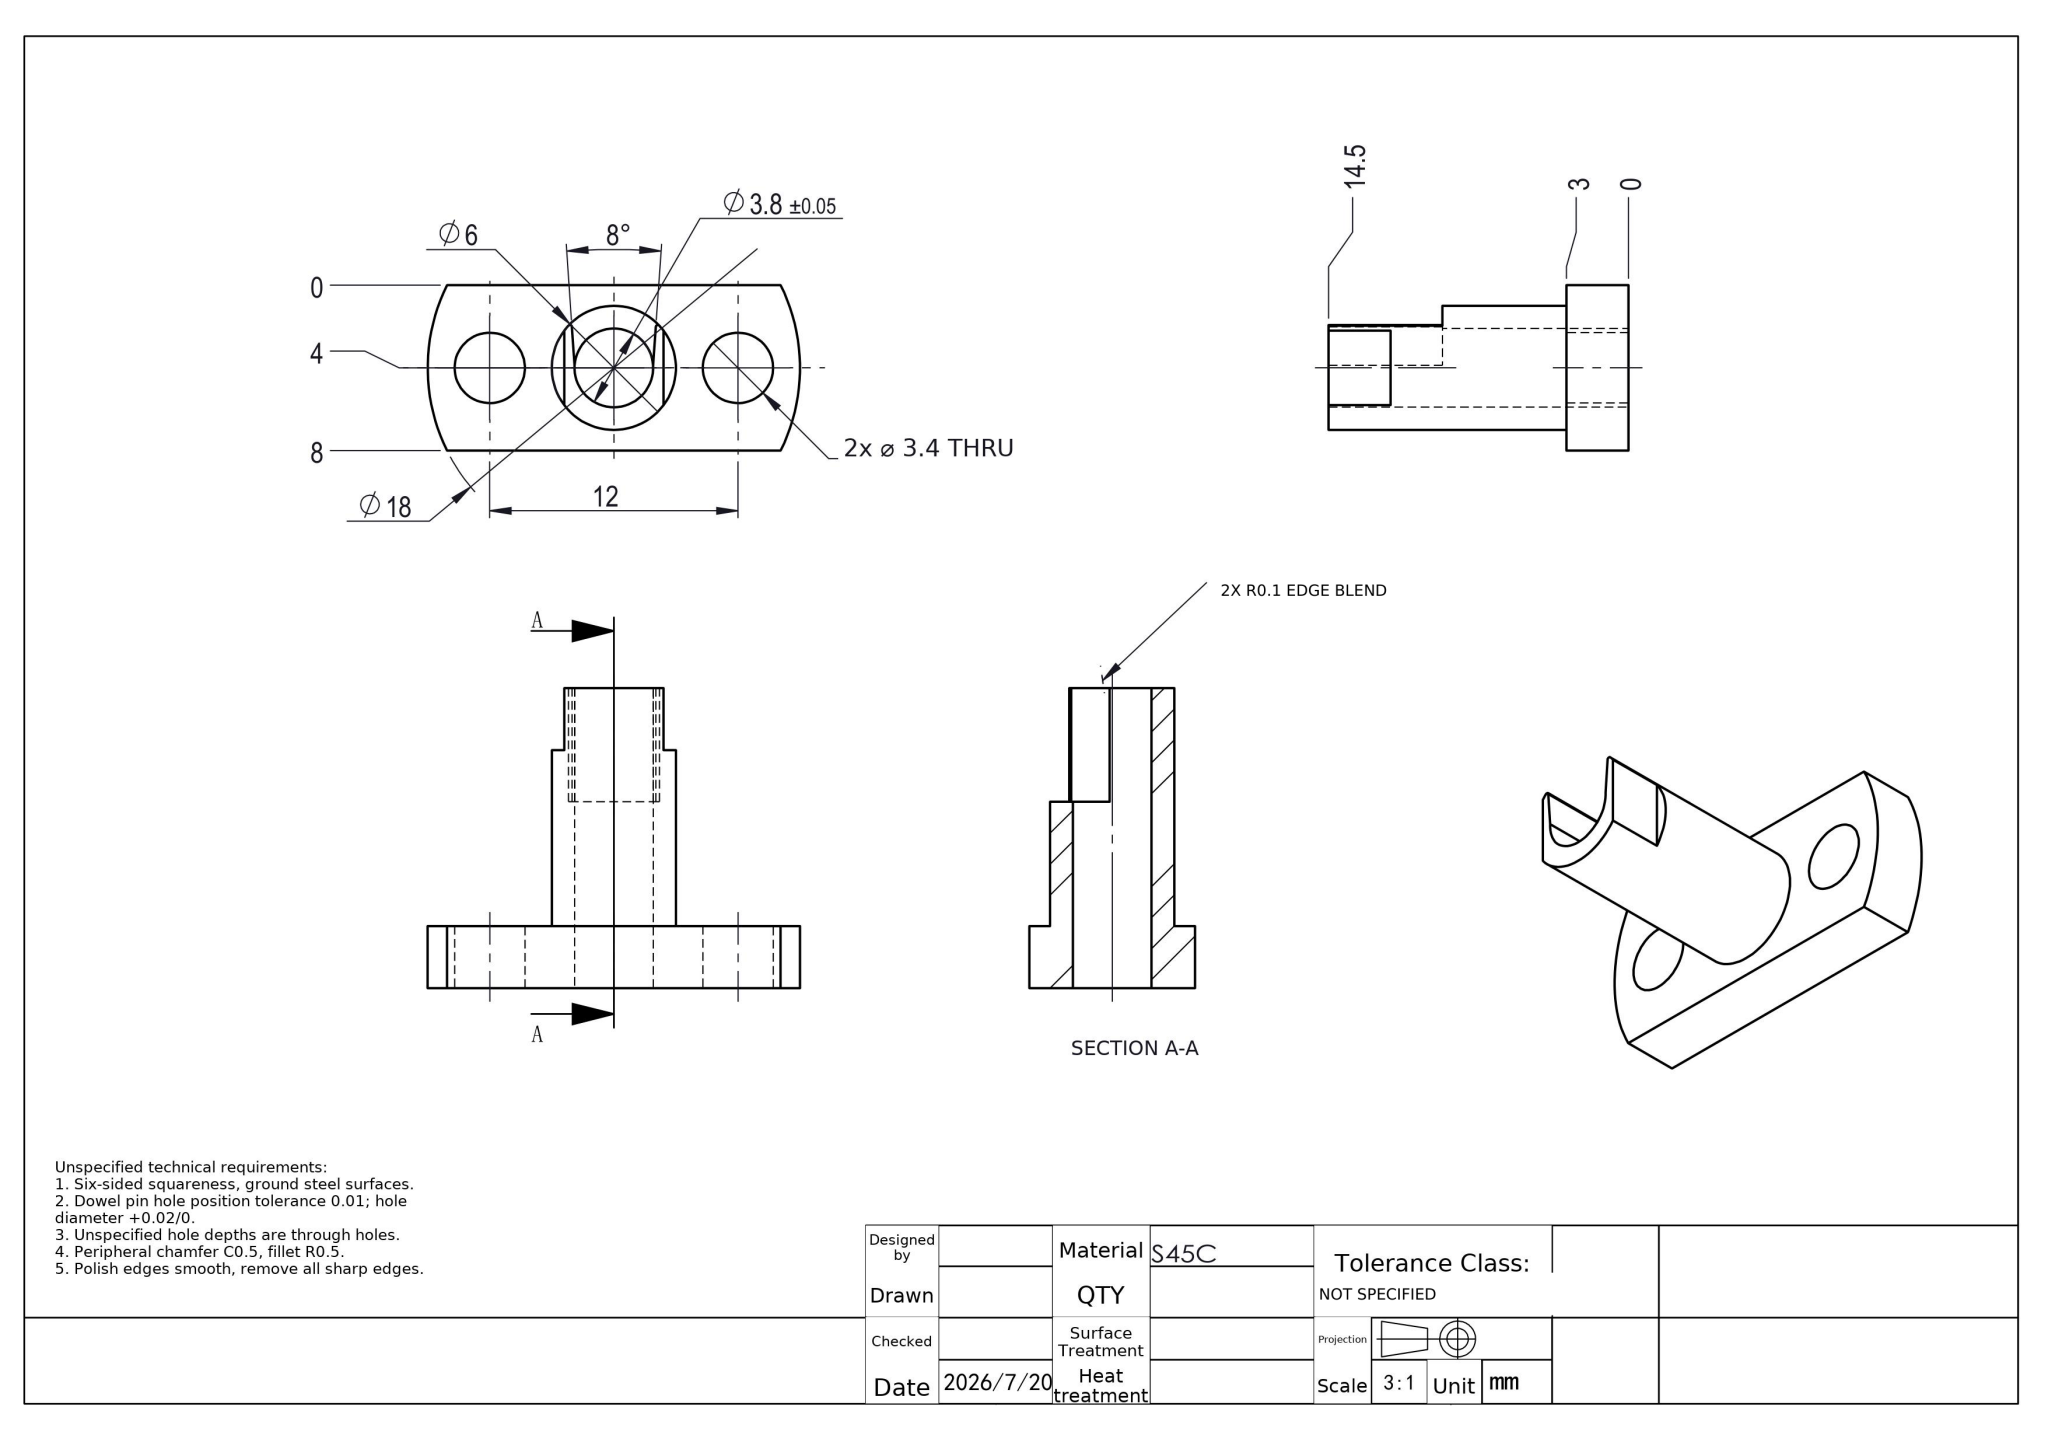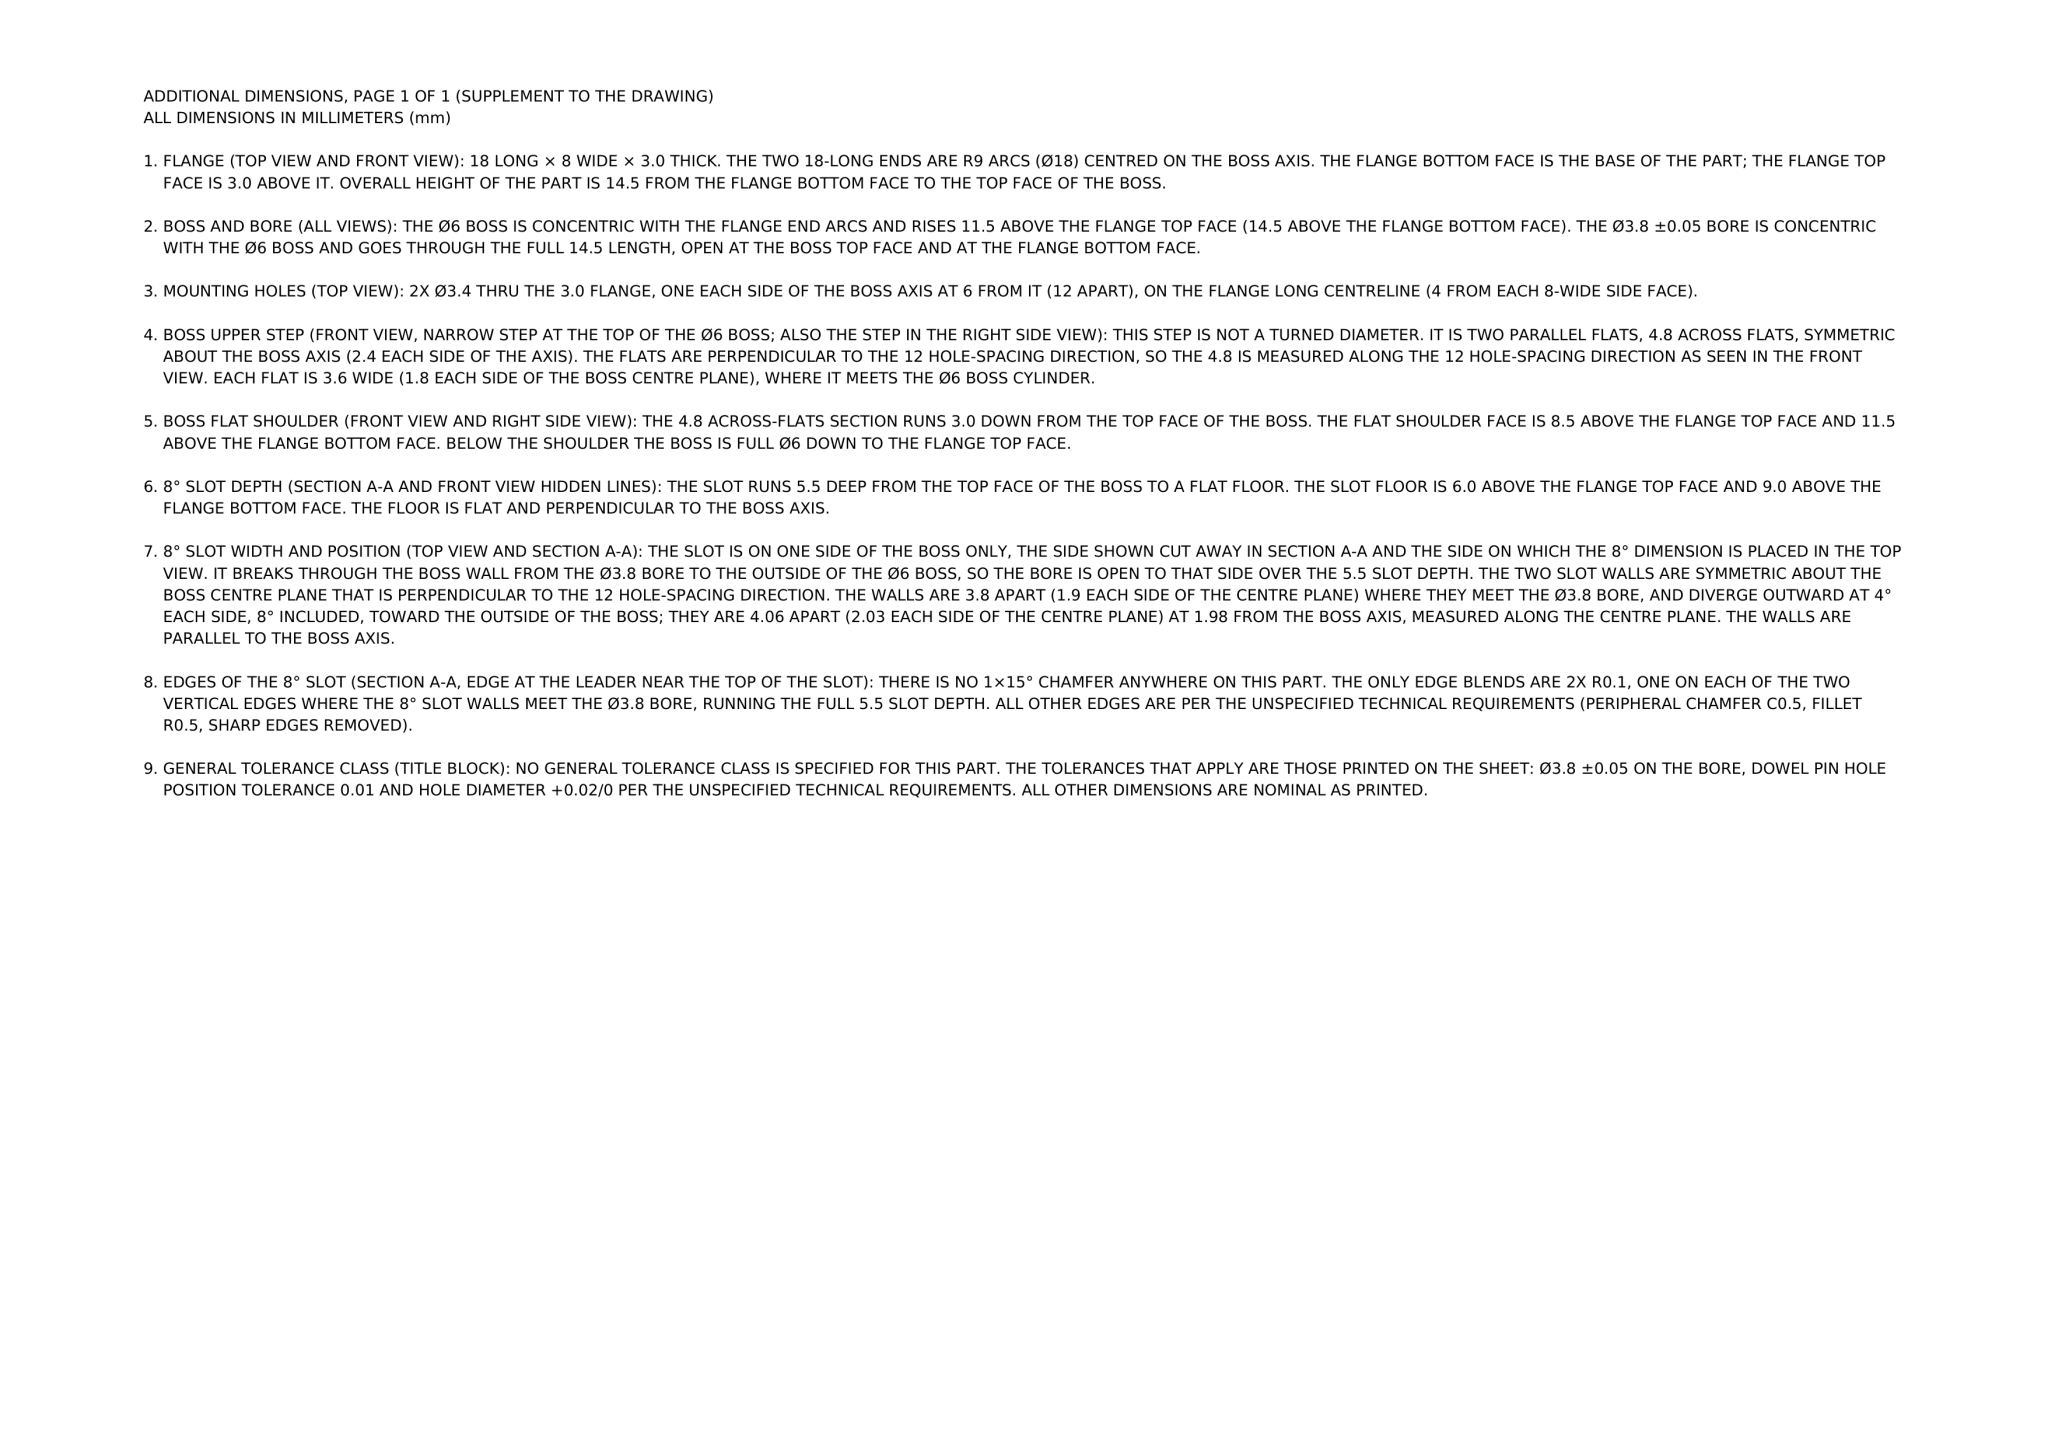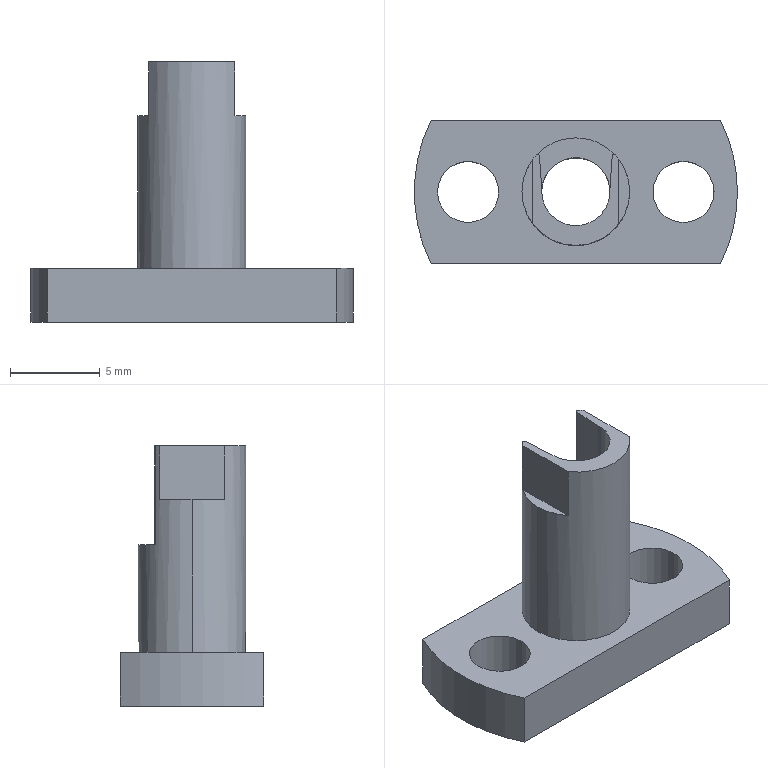Part | NX | mm | 1 solid | 25 faces | box 18 x 8 x 14.5 mm | volume 486 mm3 | cylinder 13 | plane 12 | commonest cylinder face diameters 3.4 x4 18 x3 3.8 x2 6 x2 0.2 x2
STEP:
#1=COLOUR_RGB('',0.7922,0.8196,0.9333);
#2=FILL_AREA_STYLE_COLOUR('',#1);
#3=FILL_AREA_STYLE('',(#2));
#4=SURFACE_STYLE_FILL_AREA(#3);
#5=SURFACE_SIDE_STYLE('',(#4));
#6=SURFACE_STYLE_USAGE(.BOTH.,#5);
#7=PRESENTATION_STYLE_ASSIGNMENT((#6));
#8=CARTESIAN_POINT('',(7.7,0.,0.));
#9=VERTEX_POINT('',#8);
#10=CARTESIAN_POINT('',(4.3,0.,0.));
#11=VERTEX_POINT('',#10);
#12=CARTESIAN_POINT('',(6.,0.,0.));
#13=DIRECTION('',(0.,0.,-1.));
#14=DIRECTION('',(-1.,0.,0.));
#15=AXIS2_PLACEMENT_3D('',#12,#13,#14);
#16=CIRCLE('',#15,1.7);
#17=EDGE_CURVE('',#9,#11,#16,.T.);
#18=ORIENTED_EDGE('',*,*,#17,.F.);
#19=CARTESIAN_POINT('',(7.7,0.,-3.));
#20=VERTEX_POINT('',#19);
#21=CARTESIAN_POINT('',(7.7,0.,-3.));
#22=DIRECTION('',(0.,0.,-1.));
#23=VECTOR('',#22,1000.);
#24=LINE('',#21,#23);
#25=EDGE_CURVE('',#9,#20,#24,.T.);
#26=ORIENTED_EDGE('',*,*,#25,.T.);
#27=CARTESIAN_POINT('',(4.3,0.,-3.));
#28=VERTEX_POINT('',#27);
#29=CARTESIAN_POINT('',(6.,0.,-3.));
#30=DIRECTION('',(0.,0.,-1.));
#31=DIRECTION('',(-1.,0.,0.));
#32=AXIS2_PLACEMENT_3D('',#29,#30,#31);
#33=CIRCLE('',#32,1.7);
#34=EDGE_CURVE('',#20,#28,#33,.T.);
#35=ORIENTED_EDGE('',*,*,#34,.T.);
#36=CARTESIAN_POINT('',(4.3,0.,-3.));
#37=DIRECTION('',(0.,0.,-1.));
#38=VECTOR('',#37,1000.);
#39=LINE('',#36,#38);
#40=EDGE_CURVE('',#11,#28,#39,.T.);
#41=ORIENTED_EDGE('',*,*,#40,.F.);
#42=EDGE_LOOP('',(#18,#26,#35,#41));
#43=FACE_OUTER_BOUND('',#42,.T.);
#44=CARTESIAN_POINT('',(6.,0.,-3.));
#45=DIRECTION('',(0.,0.,-1.));
#46=DIRECTION('',(-1.,0.,0.));
#47=AXIS2_PLACEMENT_3D('',#44,#45,#46);
#48=CYLINDRICAL_SURFACE('',#47,1.7);
#49=ADVANCED_FACE('',(#43),#48,.F.);
#50=CARTESIAN_POINT('',(-4.3,0.,0.));
#51=VERTEX_POINT('',#50);
#52=CARTESIAN_POINT('',(-7.7,0.,0.));
#53=VERTEX_POINT('',#52);
#54=CARTESIAN_POINT('',(-6.,0.,0.));
#55=DIRECTION('',(0.,0.,-1.));
#56=DIRECTION('',(-1.,0.,0.));
#57=AXIS2_PLACEMENT_3D('',#54,#55,#56);
#58=CIRCLE('',#57,1.7);
#59=EDGE_CURVE('',#51,#53,#58,.T.);
#60=ORIENTED_EDGE('',*,*,#59,.F.);
#61=CARTESIAN_POINT('',(-4.3,0.,-3.));
#62=VERTEX_POINT('',#61);
#63=CARTESIAN_POINT('',(-4.3,0.,-3.));
#64=DIRECTION('',(0.,0.,-1.));
#65=VECTOR('',#64,1000.);
#66=LINE('',#63,#65);
#67=EDGE_CURVE('',#51,#62,#66,.T.);
#68=ORIENTED_EDGE('',*,*,#67,.T.);
#69=CARTESIAN_POINT('',(-7.7,0.,-3.));
#70=VERTEX_POINT('',#69);
#71=CARTESIAN_POINT('',(-6.,0.,-3.));
#72=DIRECTION('',(0.,0.,-1.));
#73=DIRECTION('',(-1.,0.,0.));
#74=AXIS2_PLACEMENT_3D('',#71,#72,#73);
#75=CIRCLE('',#74,1.7);
#76=EDGE_CURVE('',#62,#70,#75,.T.);
#77=ORIENTED_EDGE('',*,*,#76,.T.);
#78=CARTESIAN_POINT('',(-7.7,0.,-3.));
#79=DIRECTION('',(0.,0.,-1.));
#80=VECTOR('',#79,1000.);
#81=LINE('',#78,#80);
#82=EDGE_CURVE('',#53,#70,#81,.T.);
#83=ORIENTED_EDGE('',*,*,#82,.F.);
#84=EDGE_LOOP('',(#60,#68,#77,#83));
#85=FACE_OUTER_BOUND('',#84,.T.);
#86=CARTESIAN_POINT('',(-6.,0.,-3.));
#87=DIRECTION('',(0.,0.,-1.));
#88=DIRECTION('',(-1.,0.,0.));
#89=AXIS2_PLACEMENT_3D('',#86,#87,#88);
#90=CYLINDRICAL_SURFACE('',#89,1.7);
#91=ADVANCED_FACE('',(#85),#90,.F.);
#92=CARTESIAN_POINT('',(9.,0.,-3.));
#93=VERTEX_POINT('',#92);
#94=CARTESIAN_POINT('',(8.062,-4.,-3.));
#95=VERTEX_POINT('',#94);
#96=CARTESIAN_POINT('',(0.,0.,-3.));
#97=DIRECTION('',(0.,0.,-1.));
#98=DIRECTION('',(-1.,0.,0.));
#99=AXIS2_PLACEMENT_3D('',#96,#97,#98);
#100=CIRCLE('',#99,9.);
#101=EDGE_CURVE('',#93,#95,#100,.T.);
#102=ORIENTED_EDGE('',*,*,#101,.F.);
#103=CARTESIAN_POINT('',(9.,0.,0.));
#104=VERTEX_POINT('',#103);
#105=CARTESIAN_POINT('',(9.,0.,-3.));
#106=DIRECTION('',(0.,0.,1.));
#107=VECTOR('',#106,1000.);
#108=LINE('',#105,#107);
#109=EDGE_CURVE('',#93,#104,#108,.T.);
#110=ORIENTED_EDGE('',*,*,#109,.T.);
#111=CARTESIAN_POINT('',(8.062,-4.,0.));
#112=VERTEX_POINT('',#111);
#113=CARTESIAN_POINT('',(0.,0.,0.));
#114=DIRECTION('',(0.,0.,-1.));
#115=DIRECTION('',(-1.,0.,0.));
#116=AXIS2_PLACEMENT_3D('',#113,#114,#115);
#117=CIRCLE('',#116,9.);
#118=EDGE_CURVE('',#104,#112,#117,.T.);
#119=ORIENTED_EDGE('',*,*,#118,.T.);
#120=CARTESIAN_POINT('',(8.062,-4.,13.));
#121=DIRECTION('',(0.,0.,-1.));
#122=VECTOR('',#121,1000.);
#123=LINE('',#120,#122);
#124=EDGE_CURVE('',#112,#95,#123,.T.);
#125=ORIENTED_EDGE('',*,*,#124,.T.);
#126=EDGE_LOOP('',(#102,#110,#119,#125));
#127=FACE_OUTER_BOUND('',#126,.T.);
#128=CARTESIAN_POINT('',(0.,0.,-3.));
#129=DIRECTION('',(0.,0.,1.));
#130=DIRECTION('',(1.,0.,0.));
#131=AXIS2_PLACEMENT_3D('',#128,#129,#130);
#132=CYLINDRICAL_SURFACE('',#131,9.);
#133=ADVANCED_FACE('',(#127),#132,.T.);
#134=CARTESIAN_POINT('',(1.9,0.,11.5));
#135=VERTEX_POINT('',#134);
#136=CARTESIAN_POINT('',(-1.9,0.,11.5));
#137=VERTEX_POINT('',#136);
#138=CARTESIAN_POINT('',(0.,0.,11.5));
#139=DIRECTION('',(0.,0.,-1.));
#140=DIRECTION('',(1.,0.,0.));
#141=AXIS2_PLACEMENT_3D('',#138,#139,#140);
#142=CIRCLE('',#141,1.9);
#143=EDGE_CURVE('',#135,#137,#142,.T.);
#144=ORIENTED_EDGE('',*,*,#143,.F.);
#145=CARTESIAN_POINT('',(1.9,0.,-3.));
#146=VERTEX_POINT('',#145);
#147=CARTESIAN_POINT('',(1.9,0.,13.));
#148=DIRECTION('',(0.,0.,-1.));
#149=VECTOR('',#148,1000.);
#150=LINE('',#147,#149);
#151=EDGE_CURVE('',#135,#146,#150,.T.);
#152=ORIENTED_EDGE('',*,*,#151,.T.);
#153=CARTESIAN_POINT('',(-1.9,0.,-3.));
#154=VERTEX_POINT('',#153);
#155=CARTESIAN_POINT('',(0.,0.,-3.));
#156=DIRECTION('',(0.,0.,-1.));
#157=DIRECTION('',(-1.,0.,0.));
#158=AXIS2_PLACEMENT_3D('',#155,#156,#157);
#159=CIRCLE('',#158,1.9);
#160=EDGE_CURVE('',#146,#154,#159,.T.);
#161=ORIENTED_EDGE('',*,*,#160,.T.);
#162=CARTESIAN_POINT('',(-1.9,0.,13.));
#163=DIRECTION('',(0.,0.,-1.));
#164=VECTOR('',#163,1000.);
#165=LINE('',#162,#164);
#166=EDGE_CURVE('',#137,#154,#165,.T.);
#167=ORIENTED_EDGE('',*,*,#166,.F.);
#168=EDGE_LOOP('',(#144,#152,#161,#167));
#169=FACE_OUTER_BOUND('',#168,.T.);
#170=CARTESIAN_POINT('',(0.,0.,13.));
#171=DIRECTION('',(0.,0.,-1.));
#172=DIRECTION('',(-1.,0.,0.));
#173=AXIS2_PLACEMENT_3D('',#170,#171,#172);
#174=CYLINDRICAL_SURFACE('',#173,1.9);
#175=ADVANCED_FACE('',(#169),#174,.F.);
#176=CARTESIAN_POINT('',(3.,0.,8.5));
#177=VERTEX_POINT('',#176);
#178=CARTESIAN_POINT('',(2.4,1.8,8.5));
#179=VERTEX_POINT('',#178);
#180=CARTESIAN_POINT('',(0.,0.,8.5));
#181=DIRECTION('',(0.,0.,1.));
#182=DIRECTION('',(-1.,0.,0.));
#183=AXIS2_PLACEMENT_3D('',#180,#181,#182);
#184=CIRCLE('',#183,3.);
#185=EDGE_CURVE('',#177,#179,#184,.T.);
#186=ORIENTED_EDGE('',*,*,#185,.F.);
#187=CARTESIAN_POINT('',(3.,0.,0.));
#188=VERTEX_POINT('',#187);
#189=CARTESIAN_POINT('',(3.,0.,13.));
#190=DIRECTION('',(0.,0.,-1.));
#191=VECTOR('',#190,1000.);
#192=LINE('',#189,#191);
#193=EDGE_CURVE('',#177,#188,#192,.T.);
#194=ORIENTED_EDGE('',*,*,#193,.T.);
#195=CARTESIAN_POINT('',(-3.,0.,0.));
#196=VERTEX_POINT('',#195);
#197=CARTESIAN_POINT('',(0.,0.,0.));
#198=DIRECTION('',(0.,0.,1.));
#199=DIRECTION('',(1.,0.,0.));
#200=AXIS2_PLACEMENT_3D('',#197,#198,#199);
#201=CIRCLE('',#200,3.);
#202=EDGE_CURVE('',#188,#196,#201,.T.);
#203=ORIENTED_EDGE('',*,*,#202,.T.);
#204=CARTESIAN_POINT('',(-3.,0.,8.5));
#205=VERTEX_POINT('',#204);
#206=CARTESIAN_POINT('',(-3.,0.,13.));
#207=DIRECTION('',(0.,0.,-1.));
#208=VECTOR('',#207,1000.);
#209=LINE('',#206,#208);
#210=EDGE_CURVE('',#205,#196,#209,.T.);
#211=ORIENTED_EDGE('',*,*,#210,.F.);
#212=CARTESIAN_POINT('',(-2.4,1.8,8.5));
#213=VERTEX_POINT('',#212);
#214=CARTESIAN_POINT('',(0.,0.,8.5));
#215=DIRECTION('',(0.,0.,1.));
#216=DIRECTION('',(1.,0.,0.));
#217=AXIS2_PLACEMENT_3D('',#214,#215,#216);
#218=CIRCLE('',#217,3.);
#219=EDGE_CURVE('',#213,#205,#218,.T.);
#220=ORIENTED_EDGE('',*,*,#219,.F.);
#221=CARTESIAN_POINT('',(-2.4,1.8,11.5));
#222=VERTEX_POINT('',#221);
#223=CARTESIAN_POINT('',(-2.4,1.8,8.5));
#224=DIRECTION('',(0.,0.,1.));
#225=VECTOR('',#224,1000.);
#226=LINE('',#223,#225);
#227=EDGE_CURVE('',#213,#222,#226,.T.);
#228=ORIENTED_EDGE('',*,*,#227,.T.);
#229=CARTESIAN_POINT('',(-2.199,2.04,11.5));
#230=VERTEX_POINT('',#229);
#231=CARTESIAN_POINT('',(0.,0.,11.5));
#232=DIRECTION('',(0.,0.,1.));
#233=DIRECTION('',(1.,0.,0.));
#234=AXIS2_PLACEMENT_3D('',#231,#232,#233);
#235=CIRCLE('',#234,3.);
#236=EDGE_CURVE('',#230,#222,#235,.T.);
#237=ORIENTED_EDGE('',*,*,#236,.F.);
#238=CARTESIAN_POINT('',(-2.199,2.04,6.));
#239=VERTEX_POINT('',#238);
#240=CARTESIAN_POINT('',(-2.199,2.04,13.));
#241=DIRECTION('',(0.,0.,-1.));
#242=VECTOR('',#241,1000.);
#243=LINE('',#240,#242);
#244=EDGE_CURVE('',#230,#239,#243,.T.);
#245=ORIENTED_EDGE('',*,*,#244,.T.);
#246=CARTESIAN_POINT('',(2.199,2.04,6.));
#247=VERTEX_POINT('',#246);
#248=CARTESIAN_POINT('',(0.,0.,6.));
#249=DIRECTION('',(0.,0.,1.));
#250=DIRECTION('',(1.,0.,0.));
#251=AXIS2_PLACEMENT_3D('',#248,#249,#250);
#252=CIRCLE('',#251,3.);
#253=EDGE_CURVE('',#247,#239,#252,.T.);
#254=ORIENTED_EDGE('',*,*,#253,.F.);
#255=CARTESIAN_POINT('',(2.199,2.04,11.5));
#256=VERTEX_POINT('',#255);
#257=CARTESIAN_POINT('',(2.199,2.04,13.));
#258=DIRECTION('',(0.,0.,1.));
#259=VECTOR('',#258,1000.);
#260=LINE('',#257,#259);
#261=EDGE_CURVE('',#247,#256,#260,.T.);
#262=ORIENTED_EDGE('',*,*,#261,.T.);
#263=CARTESIAN_POINT('',(2.4,1.8,11.5));
#264=VERTEX_POINT('',#263);
#265=CARTESIAN_POINT('',(0.,0.,11.5));
#266=DIRECTION('',(0.,0.,1.));
#267=DIRECTION('',(1.,0.,0.));
#268=AXIS2_PLACEMENT_3D('',#265,#266,#267);
#269=CIRCLE('',#268,3.);
#270=EDGE_CURVE('',#264,#256,#269,.T.);
#271=ORIENTED_EDGE('',*,*,#270,.F.);
#272=CARTESIAN_POINT('',(2.4,1.8,8.5));
#273=DIRECTION('',(0.,0.,1.));
#274=VECTOR('',#273,1000.);
#275=LINE('',#272,#274);
#276=EDGE_CURVE('',#179,#264,#275,.T.);
#277=ORIENTED_EDGE('',*,*,#276,.F.);
#278=EDGE_LOOP('',(#186,#194,#203,#211,#220,#228,#237,#245,#254,#262,#271,#277));
#279=FACE_OUTER_BOUND('',#278,.T.);
#280=CARTESIAN_POINT('',(0.,0.,13.));
#281=DIRECTION('',(0.,0.,-1.));
#282=DIRECTION('',(-1.,0.,0.));
#283=AXIS2_PLACEMENT_3D('',#280,#281,#282);
#284=CYLINDRICAL_SURFACE('',#283,3.);
#285=ADVANCED_FACE('',(#279),#284,.T.);
#286=ORIENTED_EDGE('',*,*,#193,.F.);
#287=CARTESIAN_POINT('',(2.4,-1.8,8.5));
#288=VERTEX_POINT('',#287);
#289=CARTESIAN_POINT('',(0.,0.,8.5));
#290=DIRECTION('',(0.,0.,1.));
#291=DIRECTION('',(-1.,0.,0.));
#292=AXIS2_PLACEMENT_3D('',#289,#290,#291);
#293=CIRCLE('',#292,3.);
#294=EDGE_CURVE('',#288,#177,#293,.T.);
#295=ORIENTED_EDGE('',*,*,#294,.F.);
#296=CARTESIAN_POINT('',(2.4,-1.8,11.5));
#297=VERTEX_POINT('',#296);
#298=CARTESIAN_POINT('',(2.4,-1.8,8.5));
#299=DIRECTION('',(0.,0.,1.));
#300=VECTOR('',#299,1000.);
#301=LINE('',#298,#300);
#302=EDGE_CURVE('',#288,#297,#301,.T.);
#303=ORIENTED_EDGE('',*,*,#302,.T.);
#304=CARTESIAN_POINT('',(-2.4,-1.8,11.5));
#305=VERTEX_POINT('',#304);
#306=CARTESIAN_POINT('',(0.,0.,11.5));
#307=DIRECTION('',(0.,0.,1.));
#308=DIRECTION('',(1.,0.,0.));
#309=AXIS2_PLACEMENT_3D('',#306,#307,#308);
#310=CIRCLE('',#309,3.);
#311=EDGE_CURVE('',#305,#297,#310,.T.);
#312=ORIENTED_EDGE('',*,*,#311,.F.);
#313=CARTESIAN_POINT('',(-2.4,-1.8,8.5));
#314=VERTEX_POINT('',#313);
#315=CARTESIAN_POINT('',(-2.4,-1.8,8.5));
#316=DIRECTION('',(0.,0.,1.));
#317=VECTOR('',#316,1000.);
#318=LINE('',#315,#317);
#319=EDGE_CURVE('',#314,#305,#318,.T.);
#320=ORIENTED_EDGE('',*,*,#319,.F.);
#321=CARTESIAN_POINT('',(0.,0.,8.5));
#322=DIRECTION('',(0.,0.,1.));
#323=DIRECTION('',(1.,0.,0.));
#324=AXIS2_PLACEMENT_3D('',#321,#322,#323);
#325=CIRCLE('',#324,3.);
#326=EDGE_CURVE('',#205,#314,#325,.T.);
#327=ORIENTED_EDGE('',*,*,#326,.F.);
#328=ORIENTED_EDGE('',*,*,#210,.T.);
#329=CARTESIAN_POINT('',(0.,0.,0.));
#330=DIRECTION('',(0.,0.,1.));
#331=DIRECTION('',(1.,0.,0.));
#332=AXIS2_PLACEMENT_3D('',#329,#330,#331);
#333=CIRCLE('',#332,3.);
#334=EDGE_CURVE('',#196,#188,#333,.T.);
#335=ORIENTED_EDGE('',*,*,#334,.T.);
#336=EDGE_LOOP('',(#286,#295,#303,#312,#320,#327,#328,#335));
#337=FACE_OUTER_BOUND('',#336,.T.);
#338=CARTESIAN_POINT('',(0.,0.,13.));
#339=DIRECTION('',(0.,0.,-1.));
#340=DIRECTION('',(-1.,0.,0.));
#341=AXIS2_PLACEMENT_3D('',#338,#339,#340);
#342=CYLINDRICAL_SURFACE('',#341,3.);
#343=ADVANCED_FACE('',(#337),#342,.T.);
#344=ORIENTED_EDGE('',*,*,#151,.F.);
#345=CARTESIAN_POINT('',(1.896,0.119,11.5));
#346=VERTEX_POINT('',#345);
#347=CARTESIAN_POINT('',(0.,0.,11.5));
#348=DIRECTION('',(0.,0.,-1.));
#349=DIRECTION('',(1.,0.,0.));
#350=AXIS2_PLACEMENT_3D('',#347,#348,#349);
#351=CIRCLE('',#350,1.9);
#352=EDGE_CURVE('',#346,#135,#351,.T.);
#353=ORIENTED_EDGE('',*,*,#352,.F.);
#354=CARTESIAN_POINT('',(1.896,0.119,6.));
#355=VERTEX_POINT('',#354);
#356=CARTESIAN_POINT('',(1.896,0.119,13.));
#357=DIRECTION('',(0.,0.,-1.));
#358=VECTOR('',#357,1000.);
#359=LINE('',#356,#358);
#360=EDGE_CURVE('',#346,#355,#359,.T.);
#361=ORIENTED_EDGE('',*,*,#360,.T.);
#362=CARTESIAN_POINT('',(-1.896,0.119,6.));
#363=VERTEX_POINT('',#362);
#364=CARTESIAN_POINT('',(0.,0.,6.));
#365=DIRECTION('',(0.,0.,-1.));
#366=DIRECTION('',(1.,0.,0.));
#367=AXIS2_PLACEMENT_3D('',#364,#365,#366);
#368=CIRCLE('',#367,1.9);
#369=EDGE_CURVE('',#363,#355,#368,.T.);
#370=ORIENTED_EDGE('',*,*,#369,.F.);
#371=CARTESIAN_POINT('',(-1.896,0.119,11.5));
#372=VERTEX_POINT('',#371);
#373=CARTESIAN_POINT('',(-1.896,0.119,13.));
#374=DIRECTION('',(0.,0.,1.));
#375=VECTOR('',#374,1000.);
#376=LINE('',#373,#375);
#377=EDGE_CURVE('',#363,#372,#376,.T.);
#378=ORIENTED_EDGE('',*,*,#377,.T.);
#379=CARTESIAN_POINT('',(0.,0.,11.5));
#380=DIRECTION('',(0.,0.,-1.));
#381=DIRECTION('',(1.,0.,0.));
#382=AXIS2_PLACEMENT_3D('',#379,#380,#381);
#383=CIRCLE('',#382,1.9);
#384=EDGE_CURVE('',#137,#372,#383,.T.);
#385=ORIENTED_EDGE('',*,*,#384,.F.);
#386=ORIENTED_EDGE('',*,*,#166,.T.);
#387=CARTESIAN_POINT('',(0.,0.,-3.));
#388=DIRECTION('',(0.,0.,-1.));
#389=DIRECTION('',(-1.,0.,0.));
#390=AXIS2_PLACEMENT_3D('',#387,#388,#389);
#391=CIRCLE('',#390,1.9);
#392=EDGE_CURVE('',#154,#146,#391,.T.);
#393=ORIENTED_EDGE('',*,*,#392,.T.);
#394=EDGE_LOOP('',(#344,#353,#361,#370,#378,#385,#386,#393));
#395=FACE_OUTER_BOUND('',#394,.T.);
#396=CARTESIAN_POINT('',(0.,0.,13.));
#397=DIRECTION('',(0.,0.,-1.));
#398=DIRECTION('',(-1.,0.,0.));
#399=AXIS2_PLACEMENT_3D('',#396,#397,#398);
#400=CYLINDRICAL_SURFACE('',#399,1.9);
#401=ADVANCED_FACE('',(#395),#400,.F.);
#402=CARTESIAN_POINT('',(-8.062,-4.,-3.));
#403=VERTEX_POINT('',#402);
#404=CARTESIAN_POINT('',(-8.062,4.,-3.));
#405=VERTEX_POINT('',#404);
#406=CARTESIAN_POINT('',(0.,0.,-3.));
#407=DIRECTION('',(0.,0.,-1.));
#408=DIRECTION('',(-1.,0.,0.));
#409=AXIS2_PLACEMENT_3D('',#406,#407,#408);
#410=CIRCLE('',#409,9.);
#411=EDGE_CURVE('',#403,#405,#410,.T.);
#412=ORIENTED_EDGE('',*,*,#411,.F.);
#413=CARTESIAN_POINT('',(-8.062,-4.,0.));
#414=VERTEX_POINT('',#413);
#415=CARTESIAN_POINT('',(-8.062,-4.,13.));
#416=DIRECTION('',(0.,0.,-1.));
#417=VECTOR('',#416,1000.);
#418=LINE('',#415,#417);
#419=EDGE_CURVE('',#414,#403,#418,.T.);
#420=ORIENTED_EDGE('',*,*,#419,.F.);
#421=CARTESIAN_POINT('',(-8.062,4.,0.));
#422=VERTEX_POINT('',#421);
#423=CARTESIAN_POINT('',(0.,0.,0.));
#424=DIRECTION('',(0.,0.,-1.));
#425=DIRECTION('',(-1.,0.,0.));
#426=AXIS2_PLACEMENT_3D('',#423,#424,#425);
#427=CIRCLE('',#426,9.);
#428=EDGE_CURVE('',#414,#422,#427,.T.);
#429=ORIENTED_EDGE('',*,*,#428,.T.);
#430=CARTESIAN_POINT('',(-8.062,4.,13.));
#431=DIRECTION('',(0.,0.,-1.));
#432=VECTOR('',#431,1000.);
#433=LINE('',#430,#432);
#434=EDGE_CURVE('',#422,#405,#433,.T.);
#435=ORIENTED_EDGE('',*,*,#434,.T.);
#436=EDGE_LOOP('',(#412,#420,#429,#435));
#437=FACE_OUTER_BOUND('',#436,.T.);
#438=CARTESIAN_POINT('',(0.,0.,-3.));
#439=DIRECTION('',(0.,0.,1.));
#440=DIRECTION('',(1.,0.,0.));
#441=AXIS2_PLACEMENT_3D('',#438,#439,#440);
#442=CYLINDRICAL_SURFACE('',#441,9.);
#443=ADVANCED_FACE('',(#437),#442,.T.);
#444=ORIENTED_EDGE('',*,*,#109,.F.);
#445=CARTESIAN_POINT('',(8.062,4.,-3.));
#446=VERTEX_POINT('',#445);
#447=CARTESIAN_POINT('',(0.,0.,-3.));
#448=DIRECTION('',(0.,0.,-1.));
#449=DIRECTION('',(-1.,0.,0.));
#450=AXIS2_PLACEMENT_3D('',#447,#448,#449);
#451=CIRCLE('',#450,9.);
#452=EDGE_CURVE('',#446,#93,#451,.T.);
#453=ORIENTED_EDGE('',*,*,#452,.F.);
#454=CARTESIAN_POINT('',(8.062,4.,0.));
#455=VERTEX_POINT('',#454);
#456=CARTESIAN_POINT('',(8.062,4.,13.));
#457=DIRECTION('',(0.,0.,-1.));
#458=VECTOR('',#457,1000.);
#459=LINE('',#456,#458);
#460=EDGE_CURVE('',#455,#446,#459,.T.);
#461=ORIENTED_EDGE('',*,*,#460,.F.);
#462=CARTESIAN_POINT('',(0.,0.,0.));
#463=DIRECTION('',(0.,0.,-1.));
#464=DIRECTION('',(-1.,0.,0.));
#465=AXIS2_PLACEMENT_3D('',#462,#463,#464);
#466=CIRCLE('',#465,9.);
#467=EDGE_CURVE('',#455,#104,#466,.T.);
#468=ORIENTED_EDGE('',*,*,#467,.T.);
#469=EDGE_LOOP('',(#444,#453,#461,#468));
#470=FACE_OUTER_BOUND('',#469,.T.);
#471=CARTESIAN_POINT('',(0.,0.,-3.));
#472=DIRECTION('',(0.,0.,1.));
#473=DIRECTION('',(1.,0.,0.));
#474=AXIS2_PLACEMENT_3D('',#471,#472,#473);
#475=CYLINDRICAL_SURFACE('',#474,9.);
#476=ADVANCED_FACE('',(#470),#475,.T.);
#477=CARTESIAN_POINT('',(6.,0.,-3.));
#478=DIRECTION('',(0.,0.,-1.));
#479=DIRECTION('',(-1.,0.,0.));
#480=AXIS2_PLACEMENT_3D('',#477,#478,#479);
#481=CIRCLE('',#480,1.7);
#482=EDGE_CURVE('',#28,#20,#481,.T.);
#483=ORIENTED_EDGE('',*,*,#482,.F.);
#484=ORIENTED_EDGE('',*,*,#34,.F.);
#485=EDGE_LOOP('',(#483,#484));
#486=FACE_BOUND('',#485,.T.);
#487=CARTESIAN_POINT('',(-6.,0.,-3.));
#488=DIRECTION('',(0.,0.,-1.));
#489=DIRECTION('',(-1.,0.,0.));
#490=AXIS2_PLACEMENT_3D('',#487,#488,#489);
#491=CIRCLE('',#490,1.7);
#492=EDGE_CURVE('',#70,#62,#491,.T.);
#493=ORIENTED_EDGE('',*,*,#492,.F.);
#494=ORIENTED_EDGE('',*,*,#76,.F.);
#495=EDGE_LOOP('',(#493,#494));
#496=FACE_BOUND('',#495,.T.);
#497=CARTESIAN_POINT('',(8.062,-4.,-3.));
#498=DIRECTION('',(1.,0.,0.));
#499=VECTOR('',#498,1000.);
#500=LINE('',#497,#499);
#501=EDGE_CURVE('',#403,#95,#500,.T.);
#502=ORIENTED_EDGE('',*,*,#501,.F.);
#503=ORIENTED_EDGE('',*,*,#411,.T.);
#504=CARTESIAN_POINT('',(8.062,4.,-3.));
#505=DIRECTION('',(-1.,0.,0.));
#506=VECTOR('',#505,1000.);
#507=LINE('',#504,#506);
#508=EDGE_CURVE('',#446,#405,#507,.T.);
#509=ORIENTED_EDGE('',*,*,#508,.F.);
#510=ORIENTED_EDGE('',*,*,#452,.T.);
#511=ORIENTED_EDGE('',*,*,#101,.T.);
#512=EDGE_LOOP('',(#502,#503,#509,#510,#511));
#513=FACE_OUTER_BOUND('',#512,.T.);
#514=ORIENTED_EDGE('',*,*,#392,.F.);
#515=ORIENTED_EDGE('',*,*,#160,.F.);
#516=EDGE_LOOP('',(#514,#515));
#517=FACE_BOUND('',#516,.T.);
#518=CARTESIAN_POINT('',(0.,0.,-3.));
#519=DIRECTION('',(0.,0.,-1.));
#520=DIRECTION('',(-1.,0.,0.));
#521=AXIS2_PLACEMENT_3D('',#518,#519,#520);
#522=PLANE('',#521);
#523=ADVANCED_FACE('',(#486,#496,#513,#517),#522,.T.);
#524=CARTESIAN_POINT('',(6.,0.,0.));
#525=DIRECTION('',(0.,0.,-1.));
#526=DIRECTION('',(-1.,0.,0.));
#527=AXIS2_PLACEMENT_3D('',#524,#525,#526);
#528=CIRCLE('',#527,1.7);
#529=EDGE_CURVE('',#11,#9,#528,.T.);
#530=ORIENTED_EDGE('',*,*,#529,.T.);
#531=ORIENTED_EDGE('',*,*,#17,.T.);
#532=EDGE_LOOP('',(#530,#531));
#533=FACE_BOUND('',#532,.T.);
#534=CARTESIAN_POINT('',(-6.,0.,0.));
#535=DIRECTION('',(0.,0.,-1.));
#536=DIRECTION('',(-1.,0.,0.));
#537=AXIS2_PLACEMENT_3D('',#534,#535,#536);
#538=CIRCLE('',#537,1.7);
#539=EDGE_CURVE('',#53,#51,#538,.T.);
#540=ORIENTED_EDGE('',*,*,#539,.T.);
#541=ORIENTED_EDGE('',*,*,#59,.T.);
#542=EDGE_LOOP('',(#540,#541));
#543=FACE_BOUND('',#542,.T.);
#544=ORIENTED_EDGE('',*,*,#334,.F.);
#545=ORIENTED_EDGE('',*,*,#202,.F.);
#546=EDGE_LOOP('',(#544,#545));
#547=FACE_BOUND('',#546,.T.);
#548=ORIENTED_EDGE('',*,*,#428,.F.);
#549=CARTESIAN_POINT('',(0.,-4.,0.));
#550=DIRECTION('',(1.,0.,0.));
#551=VECTOR('',#550,1000.);
#552=LINE('',#549,#551);
#553=EDGE_CURVE('',#414,#112,#552,.T.);
#554=ORIENTED_EDGE('',*,*,#553,.T.);
#555=ORIENTED_EDGE('',*,*,#118,.F.);
#556=ORIENTED_EDGE('',*,*,#467,.F.);
#557=CARTESIAN_POINT('',(0.,4.,0.));
#558=DIRECTION('',(-1.,0.,0.));
#559=VECTOR('',#558,1000.);
#560=LINE('',#557,#559);
#561=EDGE_CURVE('',#455,#422,#560,.T.);
#562=ORIENTED_EDGE('',*,*,#561,.T.);
#563=EDGE_LOOP('',(#548,#554,#555,#556,#562));
#564=FACE_OUTER_BOUND('',#563,.T.);
#565=CARTESIAN_POINT('',(0.,0.,0.));
#566=DIRECTION('',(0.,0.,-1.));
#567=DIRECTION('',(-1.,0.,0.));
#568=AXIS2_PLACEMENT_3D('',#565,#566,#567);
#569=PLANE('',#568);
#570=ADVANCED_FACE('',(#533,#543,#547,#564),#569,.F.);
#571=ORIENTED_EDGE('',*,*,#460,.T.);
#572=ORIENTED_EDGE('',*,*,#508,.T.);
#573=ORIENTED_EDGE('',*,*,#434,.F.);
#574=ORIENTED_EDGE('',*,*,#561,.F.);
#575=EDGE_LOOP('',(#571,#572,#573,#574));
#576=FACE_OUTER_BOUND('',#575,.T.);
#577=CARTESIAN_POINT('',(8.062,4.,13.));
#578=DIRECTION('',(0.,-1.,0.));
#579=DIRECTION('',(0.,0.,-1.));
#580=AXIS2_PLACEMENT_3D('',#577,#578,#579);
#581=PLANE('',#580);
#582=ADVANCED_FACE('',(#576),#581,.F.);
#583=ORIENTED_EDGE('',*,*,#419,.T.);
#584=ORIENTED_EDGE('',*,*,#501,.T.);
#585=ORIENTED_EDGE('',*,*,#124,.F.);
#586=ORIENTED_EDGE('',*,*,#553,.F.);
#587=EDGE_LOOP('',(#583,#584,#585,#586));
#588=FACE_OUTER_BOUND('',#587,.T.);
#589=CARTESIAN_POINT('',(8.062,-4.,13.));
#590=DIRECTION('',(0.,1.,0.));
#591=DIRECTION('',(0.,0.,1.));
#592=AXIS2_PLACEMENT_3D('',#589,#590,#591);
#593=PLANE('',#592);
#594=ADVANCED_FACE('',(#588),#593,.F.);
#595=ORIENTED_EDGE('',*,*,#67,.F.);
#596=ORIENTED_EDGE('',*,*,#539,.F.);
#597=ORIENTED_EDGE('',*,*,#82,.T.);
#598=ORIENTED_EDGE('',*,*,#492,.T.);
#599=EDGE_LOOP('',(#595,#596,#597,#598));
#600=FACE_OUTER_BOUND('',#599,.T.);
#601=CARTESIAN_POINT('',(-6.,0.,-3.));
#602=DIRECTION('',(0.,0.,-1.));
#603=DIRECTION('',(-1.,0.,0.));
#604=AXIS2_PLACEMENT_3D('',#601,#602,#603);
#605=CYLINDRICAL_SURFACE('',#604,1.7);
#606=ADVANCED_FACE('',(#600),#605,.F.);
#607=ORIENTED_EDGE('',*,*,#25,.F.);
#608=ORIENTED_EDGE('',*,*,#529,.F.);
#609=ORIENTED_EDGE('',*,*,#40,.T.);
#610=ORIENTED_EDGE('',*,*,#482,.T.);
#611=EDGE_LOOP('',(#607,#608,#609,#610));
#612=FACE_OUTER_BOUND('',#611,.T.);
#613=CARTESIAN_POINT('',(6.,0.,-3.));
#614=DIRECTION('',(0.,0.,-1.));
#615=DIRECTION('',(-1.,0.,0.));
#616=AXIS2_PLACEMENT_3D('',#613,#614,#615);
#617=CYLINDRICAL_SURFACE('',#616,1.7);
#618=ADVANCED_FACE('',(#612),#617,.F.);
#619=CARTESIAN_POINT('',(2.4,1.8,11.5));
#620=DIRECTION('',(0.,-1.,0.));
#621=VECTOR('',#620,1000.);
#622=LINE('',#619,#621);
#623=EDGE_CURVE('',#264,#297,#622,.T.);
#624=ORIENTED_EDGE('',*,*,#623,.F.);
#625=ORIENTED_EDGE('',*,*,#270,.T.);
#626=CARTESIAN_POINT('',(2.026,1.979,11.5));
#627=VERTEX_POINT('',#626);
#628=CARTESIAN_POINT('',(2.126,1.972,11.5));
#629=DIRECTION('',(0.,0.,1.));
#630=DIRECTION('',(1.,0.,0.));
#631=AXIS2_PLACEMENT_3D('',#628,#629,#630);
#632=CIRCLE('',#631,0.1);
#633=EDGE_CURVE('',#256,#627,#632,.T.);
#634=ORIENTED_EDGE('',*,*,#633,.T.);
#635=CARTESIAN_POINT('',(1.879,-0.1314,11.5));
#636=DIRECTION('',(0.06976,0.9976,0.));
#637=VECTOR('',#636,1000.);
#638=LINE('',#635,#637);
#639=EDGE_CURVE('',#346,#627,#638,.T.);
#640=ORIENTED_EDGE('',*,*,#639,.F.);
#641=ORIENTED_EDGE('',*,*,#352,.T.);
#642=ORIENTED_EDGE('',*,*,#143,.T.);
#643=ORIENTED_EDGE('',*,*,#384,.T.);
#644=CARTESIAN_POINT('',(-2.026,1.979,11.5));
#645=VERTEX_POINT('',#644);
#646=CARTESIAN_POINT('',(-1.879,-0.1314,11.5));
#647=DIRECTION('',(0.06976,-0.9976,0.));
#648=VECTOR('',#647,1000.);
#649=LINE('',#646,#648);
#650=EDGE_CURVE('',#645,#372,#649,.T.);
#651=ORIENTED_EDGE('',*,*,#650,.F.);
#652=CARTESIAN_POINT('',(-2.126,1.972,11.5));
#653=DIRECTION('',(0.,0.,1.));
#654=DIRECTION('',(1.,0.,0.));
#655=AXIS2_PLACEMENT_3D('',#652,#653,#654);
#656=CIRCLE('',#655,0.1);
#657=EDGE_CURVE('',#645,#230,#656,.T.);
#658=ORIENTED_EDGE('',*,*,#657,.T.);
#659=ORIENTED_EDGE('',*,*,#236,.T.);
#660=CARTESIAN_POINT('',(-2.4,1.8,11.5));
#661=DIRECTION('',(0.,1.,0.));
#662=VECTOR('',#661,1000.);
#663=LINE('',#660,#662);
#664=EDGE_CURVE('',#305,#222,#663,.T.);
#665=ORIENTED_EDGE('',*,*,#664,.F.);
#666=ORIENTED_EDGE('',*,*,#311,.T.);
#667=EDGE_LOOP('',(#624,#625,#634,#640,#641,#642,#643,#651,#658,#659,#665,#666));
#668=FACE_OUTER_BOUND('',#667,.T.);
#669=CARTESIAN_POINT('',(0.,0.,11.5));
#670=DIRECTION('',(0.,0.,1.));
#671=DIRECTION('',(1.,0.,0.));
#672=AXIS2_PLACEMENT_3D('',#669,#670,#671);
#673=PLANE('',#672);
#674=ADVANCED_FACE('',(#668),#673,.T.);
#675=ORIENTED_EDGE('',*,*,#253,.T.);
#676=CARTESIAN_POINT('',(-2.026,1.979,6.));
#677=VERTEX_POINT('',#676);
#678=CARTESIAN_POINT('',(-2.126,1.972,6.));
#679=DIRECTION('',(0.,0.,-1.));
#680=DIRECTION('',(1.,0.,0.));
#681=AXIS2_PLACEMENT_3D('',#678,#679,#680);
#682=CIRCLE('',#681,0.1);
#683=EDGE_CURVE('',#239,#677,#682,.T.);
#684=ORIENTED_EDGE('',*,*,#683,.T.);
#685=CARTESIAN_POINT('',(-1.861,-0.3818,6.));
#686=DIRECTION('',(0.06976,-0.9976,0.));
#687=VECTOR('',#686,1000.);
#688=LINE('',#685,#687);
#689=EDGE_CURVE('',#677,#363,#688,.T.);
#690=ORIENTED_EDGE('',*,*,#689,.T.);
#691=ORIENTED_EDGE('',*,*,#369,.T.);
#692=CARTESIAN_POINT('',(2.026,1.979,6.));
#693=VERTEX_POINT('',#692);
#694=CARTESIAN_POINT('',(1.861,-0.3818,6.));
#695=DIRECTION('',(0.06976,0.9976,0.));
#696=VECTOR('',#695,1000.);
#697=LINE('',#694,#696);
#698=EDGE_CURVE('',#355,#693,#697,.T.);
#699=ORIENTED_EDGE('',*,*,#698,.T.);
#700=CARTESIAN_POINT('',(2.126,1.972,6.));
#701=DIRECTION('',(0.,0.,-1.));
#702=DIRECTION('',(1.,0.,0.));
#703=AXIS2_PLACEMENT_3D('',#700,#701,#702);
#704=CIRCLE('',#703,0.1);
#705=EDGE_CURVE('',#693,#247,#704,.T.);
#706=ORIENTED_EDGE('',*,*,#705,.T.);
#707=EDGE_LOOP('',(#675,#684,#690,#691,#699,#706));
#708=FACE_OUTER_BOUND('',#707,.T.);
#709=CARTESIAN_POINT('',(0.,0.,6.));
#710=DIRECTION('',(0.,0.,1.));
#711=DIRECTION('',(1.,0.,0.));
#712=AXIS2_PLACEMENT_3D('',#709,#710,#711);
#713=PLANE('',#712);
#714=ADVANCED_FACE('',(#708),#713,.T.);
#715=ORIENTED_EDGE('',*,*,#689,.F.);
#716=CARTESIAN_POINT('',(-2.026,1.979,6.));
#717=DIRECTION('',(0.,0.,1.));
#718=VECTOR('',#717,1000.);
#719=LINE('',#716,#718);
#720=EDGE_CURVE('',#677,#645,#719,.T.);
#721=ORIENTED_EDGE('',*,*,#720,.T.);
#722=ORIENTED_EDGE('',*,*,#650,.T.);
#723=ORIENTED_EDGE('',*,*,#377,.F.);
#724=EDGE_LOOP('',(#715,#721,#722,#723));
#725=FACE_OUTER_BOUND('',#724,.T.);
#726=CARTESIAN_POINT('',(-1.861,-0.3818,6.));
#727=DIRECTION('',(-0.9976,-0.06976,0.));
#728=DIRECTION('',(0.06976,-0.9976,0.));
#729=AXIS2_PLACEMENT_3D('',#726,#727,#728);
#730=PLANE('',#729);
#731=ADVANCED_FACE('',(#725),#730,.F.);
#732=ORIENTED_EDGE('',*,*,#639,.T.);
#733=CARTESIAN_POINT('',(2.026,1.979,6.));
#734=DIRECTION('',(0.,0.,-1.));
#735=VECTOR('',#734,1000.);
#736=LINE('',#733,#735);
#737=EDGE_CURVE('',#627,#693,#736,.T.);
#738=ORIENTED_EDGE('',*,*,#737,.T.);
#739=ORIENTED_EDGE('',*,*,#698,.F.);
#740=ORIENTED_EDGE('',*,*,#360,.F.);
#741=EDGE_LOOP('',(#732,#738,#739,#740));
#742=FACE_OUTER_BOUND('',#741,.T.);
#743=CARTESIAN_POINT('',(1.861,-0.3818,6.));
#744=DIRECTION('',(0.9976,-0.06976,0.));
#745=DIRECTION('',(0.06976,0.9976,0.));
#746=AXIS2_PLACEMENT_3D('',#743,#744,#745);
#747=PLANE('',#746);
#748=ADVANCED_FACE('',(#742),#747,.F.);
#749=ORIENTED_EDGE('',*,*,#705,.F.);
#750=ORIENTED_EDGE('',*,*,#737,.F.);
#751=ORIENTED_EDGE('',*,*,#633,.F.);
#752=ORIENTED_EDGE('',*,*,#261,.F.);
#753=EDGE_LOOP('',(#749,#750,#751,#752));
#754=FACE_OUTER_BOUND('',#753,.T.);
#755=CARTESIAN_POINT('',(2.126,1.972,13.));
#756=DIRECTION('',(0.,0.,-1.));
#757=DIRECTION('',(-1.,0.,0.));
#758=AXIS2_PLACEMENT_3D('',#755,#756,#757);
#759=CYLINDRICAL_SURFACE('',#758,0.1);
#760=ADVANCED_FACE('',(#754),#759,.T.);
#761=ORIENTED_EDGE('',*,*,#657,.F.);
#762=ORIENTED_EDGE('',*,*,#720,.F.);
#763=ORIENTED_EDGE('',*,*,#683,.F.);
#764=ORIENTED_EDGE('',*,*,#244,.F.);
#765=EDGE_LOOP('',(#761,#762,#763,#764));
#766=FACE_OUTER_BOUND('',#765,.T.);
#767=CARTESIAN_POINT('',(-2.126,1.972,13.));
#768=DIRECTION('',(0.,0.,-1.));
#769=DIRECTION('',(-1.,0.,0.));
#770=AXIS2_PLACEMENT_3D('',#767,#768,#769);
#771=CYLINDRICAL_SURFACE('',#770,0.1);
#772=ADVANCED_FACE('',(#766),#771,.T.);
#773=ORIENTED_EDGE('',*,*,#664,.T.);
#774=ORIENTED_EDGE('',*,*,#227,.F.);
#775=CARTESIAN_POINT('',(-2.4,1.8,8.5));
#776=DIRECTION('',(0.,1.,0.));
#777=VECTOR('',#776,1000.);
#778=LINE('',#775,#777);
#779=EDGE_CURVE('',#314,#213,#778,.T.);
#780=ORIENTED_EDGE('',*,*,#779,.F.);
#781=ORIENTED_EDGE('',*,*,#319,.T.);
#782=EDGE_LOOP('',(#773,#774,#780,#781));
#783=FACE_OUTER_BOUND('',#782,.T.);
#784=CARTESIAN_POINT('',(-2.4,1.8,8.5));
#785=DIRECTION('',(1.,0.,0.));
#786=DIRECTION('',(0.,0.,-1.));
#787=AXIS2_PLACEMENT_3D('',#784,#785,#786);
#788=PLANE('',#787);
#789=ADVANCED_FACE('',(#783),#788,.F.);
#790=ORIENTED_EDGE('',*,*,#219,.T.);
#791=ORIENTED_EDGE('',*,*,#326,.T.);
#792=ORIENTED_EDGE('',*,*,#779,.T.);
#793=EDGE_LOOP('',(#790,#791,#792));
#794=FACE_OUTER_BOUND('',#793,.T.);
#795=CARTESIAN_POINT('',(0.,0.,8.5));
#796=DIRECTION('',(0.,0.,1.));
#797=DIRECTION('',(1.,0.,0.));
#798=AXIS2_PLACEMENT_3D('',#795,#796,#797);
#799=PLANE('',#798);
#800=ADVANCED_FACE('',(#794),#799,.T.);
#801=ORIENTED_EDGE('',*,*,#623,.T.);
#802=ORIENTED_EDGE('',*,*,#302,.F.);
#803=CARTESIAN_POINT('',(2.4,1.8,8.5));
#804=DIRECTION('',(0.,-1.,0.));
#805=VECTOR('',#804,1000.);
#806=LINE('',#803,#805);
#807=EDGE_CURVE('',#179,#288,#806,.T.);
#808=ORIENTED_EDGE('',*,*,#807,.F.);
#809=ORIENTED_EDGE('',*,*,#276,.T.);
#810=EDGE_LOOP('',(#801,#802,#808,#809));
#811=FACE_OUTER_BOUND('',#810,.T.);
#812=CARTESIAN_POINT('',(2.4,1.8,8.5));
#813=DIRECTION('',(-1.,0.,0.));
#814=DIRECTION('',(0.,0.,1.));
#815=AXIS2_PLACEMENT_3D('',#812,#813,#814);
#816=PLANE('',#815);
#817=ADVANCED_FACE('',(#811),#816,.F.);
#818=ORIENTED_EDGE('',*,*,#294,.T.);
#819=ORIENTED_EDGE('',*,*,#185,.T.);
#820=ORIENTED_EDGE('',*,*,#807,.T.);
#821=EDGE_LOOP('',(#818,#819,#820));
#822=FACE_OUTER_BOUND('',#821,.T.);
#823=CARTESIAN_POINT('',(0.,0.,8.5));
#824=DIRECTION('',(0.,0.,-1.));
#825=DIRECTION('',(-1.,0.,0.));
#826=AXIS2_PLACEMENT_3D('',#823,#824,#825);
#827=PLANE('',#826);
#828=ADVANCED_FACE('',(#822),#827,.F.);
#829=CLOSED_SHELL('',(#49,#91,#133,#175,#285,#343,#401,#443,#476,#523,#570,#582,#594,#606,#618,#674,#714,#731,#748,#760,#772,#789,#800,#817,#828));
#830=MANIFOLD_SOLID_BREP('',#829);
#831=STYLED_ITEM('',(#7),#830);
#832=PRESENTATION_LAYER_ASSIGNMENT('','',(#831));
#833=CARTESIAN_POINT('',(0.,0.,0.));
#834=DIRECTION('',(0.,0.,1.));
#835=DIRECTION('',(1.,0.,0.));
#836=AXIS2_PLACEMENT_3D('',#833,#834,#835);
#837=(LENGTH_UNIT()NAMED_UNIT(*)SI_UNIT(.MILLI.,.METRE.));
#838=UNCERTAINTY_MEASURE_WITH_UNIT(LENGTH_MEASURE(0.00001),#837,'','');
#839=(NAMED_UNIT(*)PLANE_ANGLE_UNIT()SI_UNIT($,.RADIAN.));
#840=(NAMED_UNIT(*)SI_UNIT($,.STERADIAN.)SOLID_ANGLE_UNIT());
#841=(GEOMETRIC_REPRESENTATION_CONTEXT(3)GLOBAL_UNCERTAINTY_ASSIGNED_CONTEXT((#838))GLOBAL_UNIT_ASSIGNED_CONTEXT((#837,#839,#840))REPRESENTATION_CONTEXT('',''));
#842=ADVANCED_BREP_SHAPE_REPRESENTATION('',(#830,#836),#841);
#843=(LENGTH_UNIT()NAMED_UNIT(*)SI_UNIT(.MILLI.,.METRE.));
#844=UNCERTAINTY_MEASURE_WITH_UNIT(LENGTH_MEASURE(0.00001),#843,'','');
#845=(NAMED_UNIT(*)PLANE_ANGLE_UNIT()SI_UNIT($,.RADIAN.));
#846=(NAMED_UNIT(*)SI_UNIT($,.STERADIAN.)SOLID_ANGLE_UNIT());
#847=(GEOMETRIC_REPRESENTATION_CONTEXT(3)GLOBAL_UNCERTAINTY_ASSIGNED_CONTEXT((#844))GLOBAL_UNIT_ASSIGNED_CONTEXT((#843,#845,#846))REPRESENTATION_CONTEXT('',''));
#848=MECHANICAL_DESIGN_GEOMETRIC_PRESENTATION_REPRESENTATION('',(#831),#847);